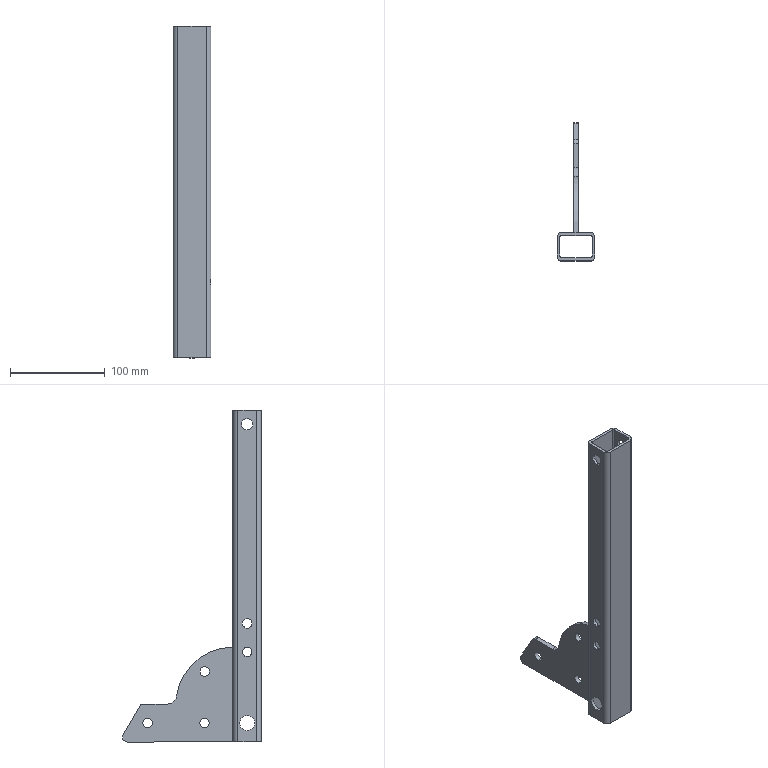Component | SolidWorks | SeederBracket-1 | 2 solids | 57 faces | box 40 x 146.34 x 350 mm | volume 158556 mm3 | cylinder 37 | plane 20 | commonest cylinder face diameters 10 x19 4 x6 16 x4 12 x4 24.2 x2 20 x1 120 x1
build123d program:
from build123d import *

# Parameters (mm, degrees)
BOSS_EXTRUDE1_DEPTH  = 175
SKETCH2_R            = 6
CUT_EXTRUDE1_2_DEPTH = 181.139
SKETCH3_R            = 8
CUT_EXTRUDE2_DEPTH   = 400
BOSS_EXTRUDE2_DEPTH  = 2.5
SKETCH6_R            = 5
CUT_EXTRUDE3_DEPTH   = 5
SKETCH7_R            = 5
CUT_EXTRUDE4_DEPTH   = 223.43
SKETCH1_R            = 12.1
CUT_EXTRUDE1_DEPTH   = 5.1


with BuildPart() as part:
    # Sketch1_2 → Boss-Extrude1 (new, symmetric)
    with BuildSketch(Plane.XY):
        with BuildLine():
            Line((-15, -15), (15, -15))
            ThreePointArc((15, -15), (18.536, -13.536), (20, -10))
            Line((20, -10), (20, 10))
            ThreePointArc((20, 10), (18.536, 13.536), (15, 15))
            Line((15, 15), (-15, 15))
            ThreePointArc((-15, 15), (-18.536, 13.536), (-20, 10))
            Line((-20, 10), (-20, -10))
            ThreePointArc((-20, -10), (-18.536, -13.536), (-15, -15))
        make_face()
        with BuildLine():
            Line((-15, 12), (15, 12))
            ThreePointArc((15, 12), (16.414, 11.414), (17, 10))
            Line((17, 10), (17, -10))
            ThreePointArc((17, -10), (16.414, -11.414), (15, -12))
            Line((15, -12), (-15, -12))
            ThreePointArc((-15, -12), (-16.414, -11.414), (-17, -10))
            Line((-17, -10), (-17, 10))
            ThreePointArc((-17, 10), (-16.414, 11.414), (-15, 12))
        make_face(mode=Mode.SUBTRACT)
    extrude(amount=BOSS_EXTRUDE1_DEPTH, both=True)

    # Sketch2 → Cut-Extrude1_2 (cut, through all)
    with BuildSketch(Plane(origin=(20, 0, 0), x_dir=(0, 0, -1), z_dir=(1, 0, 0))):
        with Locations((-160, 0)):
            Circle(SKETCH2_R)
    extrude(amount=-CUT_EXTRUDE1_2_DEPTH, mode=Mode.SUBTRACT)

    # Sketch3 → Cut-Extrude2 (cut)
    with BuildSketch(Plane(origin=(20, 0, 0), x_dir=(0, 0, -1), z_dir=(1, 0, 0))):
        with Locations((155, 0)):
            Circle(SKETCH3_R)
    extrude(amount=-CUT_EXTRUDE2_DEPTH, mode=Mode.SUBTRACT)

    # Sketch7 → Cut-Extrude4 (cut, through all)
    with BuildSketch(Plane(origin=(20, 0, 0), x_dir=(0, 0, -1), z_dir=(1, 0, 0))):
        with Locations((80, 0)):
            Circle(SKETCH7_R)
        with Locations((50, 0)):
            Circle(SKETCH7_R)
    extrude(amount=-CUT_EXTRUDE4_DEPTH, mode=Mode.SUBTRACT)

    # Sketch1 → Cut-Extrude1 (cut)
    with BuildSketch(Plane(origin=(20, 0, 0), x_dir=(0, 0, -1), z_dir=(1, 0, 0))):
        with Locations((94.684, 0)):
            Circle(SKETCH1_R)
    extrude(amount=-CUT_EXTRUDE1_DEPTH, mode=Mode.SUBTRACT)


with BuildPart() as body_2:
    # Sketch5 → Boss-Extrude2 (new, symmetric)
    with BuildSketch(Plane(origin=(0, 0, 0), x_dir=(0, 0, -1), z_dir=(1, 0, 0))):
        with BuildLine():
            Line((175, 15), (175, 126.34))
            ThreePointArc((175, 126.34), (172.5, 130.67), (167.5, 130.67))
            Line((167.5, 130.67), (137.5, 113.349))
            ThreePointArc((137.5, 113.349), (135.67, 111.519), (135, 109.019))
            Line((135, 109.019), (135, 84.282))
            ThreePointArc((135, 84.282), (132.559, 77.735), (126.429, 74.385))
            ThreePointArc((126.429, 74.385), (89.644, 54.279), (75, 15))
            Line((75, 15), (175, 15))
        make_face()
    extrude(amount=BOSS_EXTRUDE2_DEPTH, both=True)

    # Sketch6 → Cut-Extrude3 (cut)
    with BuildSketch(Plane(origin=(2.5, 0, 0), x_dir=(0, 0, -1), z_dir=(1, 0, 0))):
        with Locations((155, 105)):
            Circle(SKETCH6_R)
        with Locations((155, 45)):
            Circle(SKETCH6_R)
        with Locations((100.714, 44.692)):
            Circle(SKETCH6_R)
    extrude(amount=-CUT_EXTRUDE3_DEPTH, mode=Mode.SUBTRACT)


solid = Compound([part.part, body_2.part])

# Placed as in the assembly
solid = solid.moved(Location((0, -105, -157.5), (0, 0, 0)))